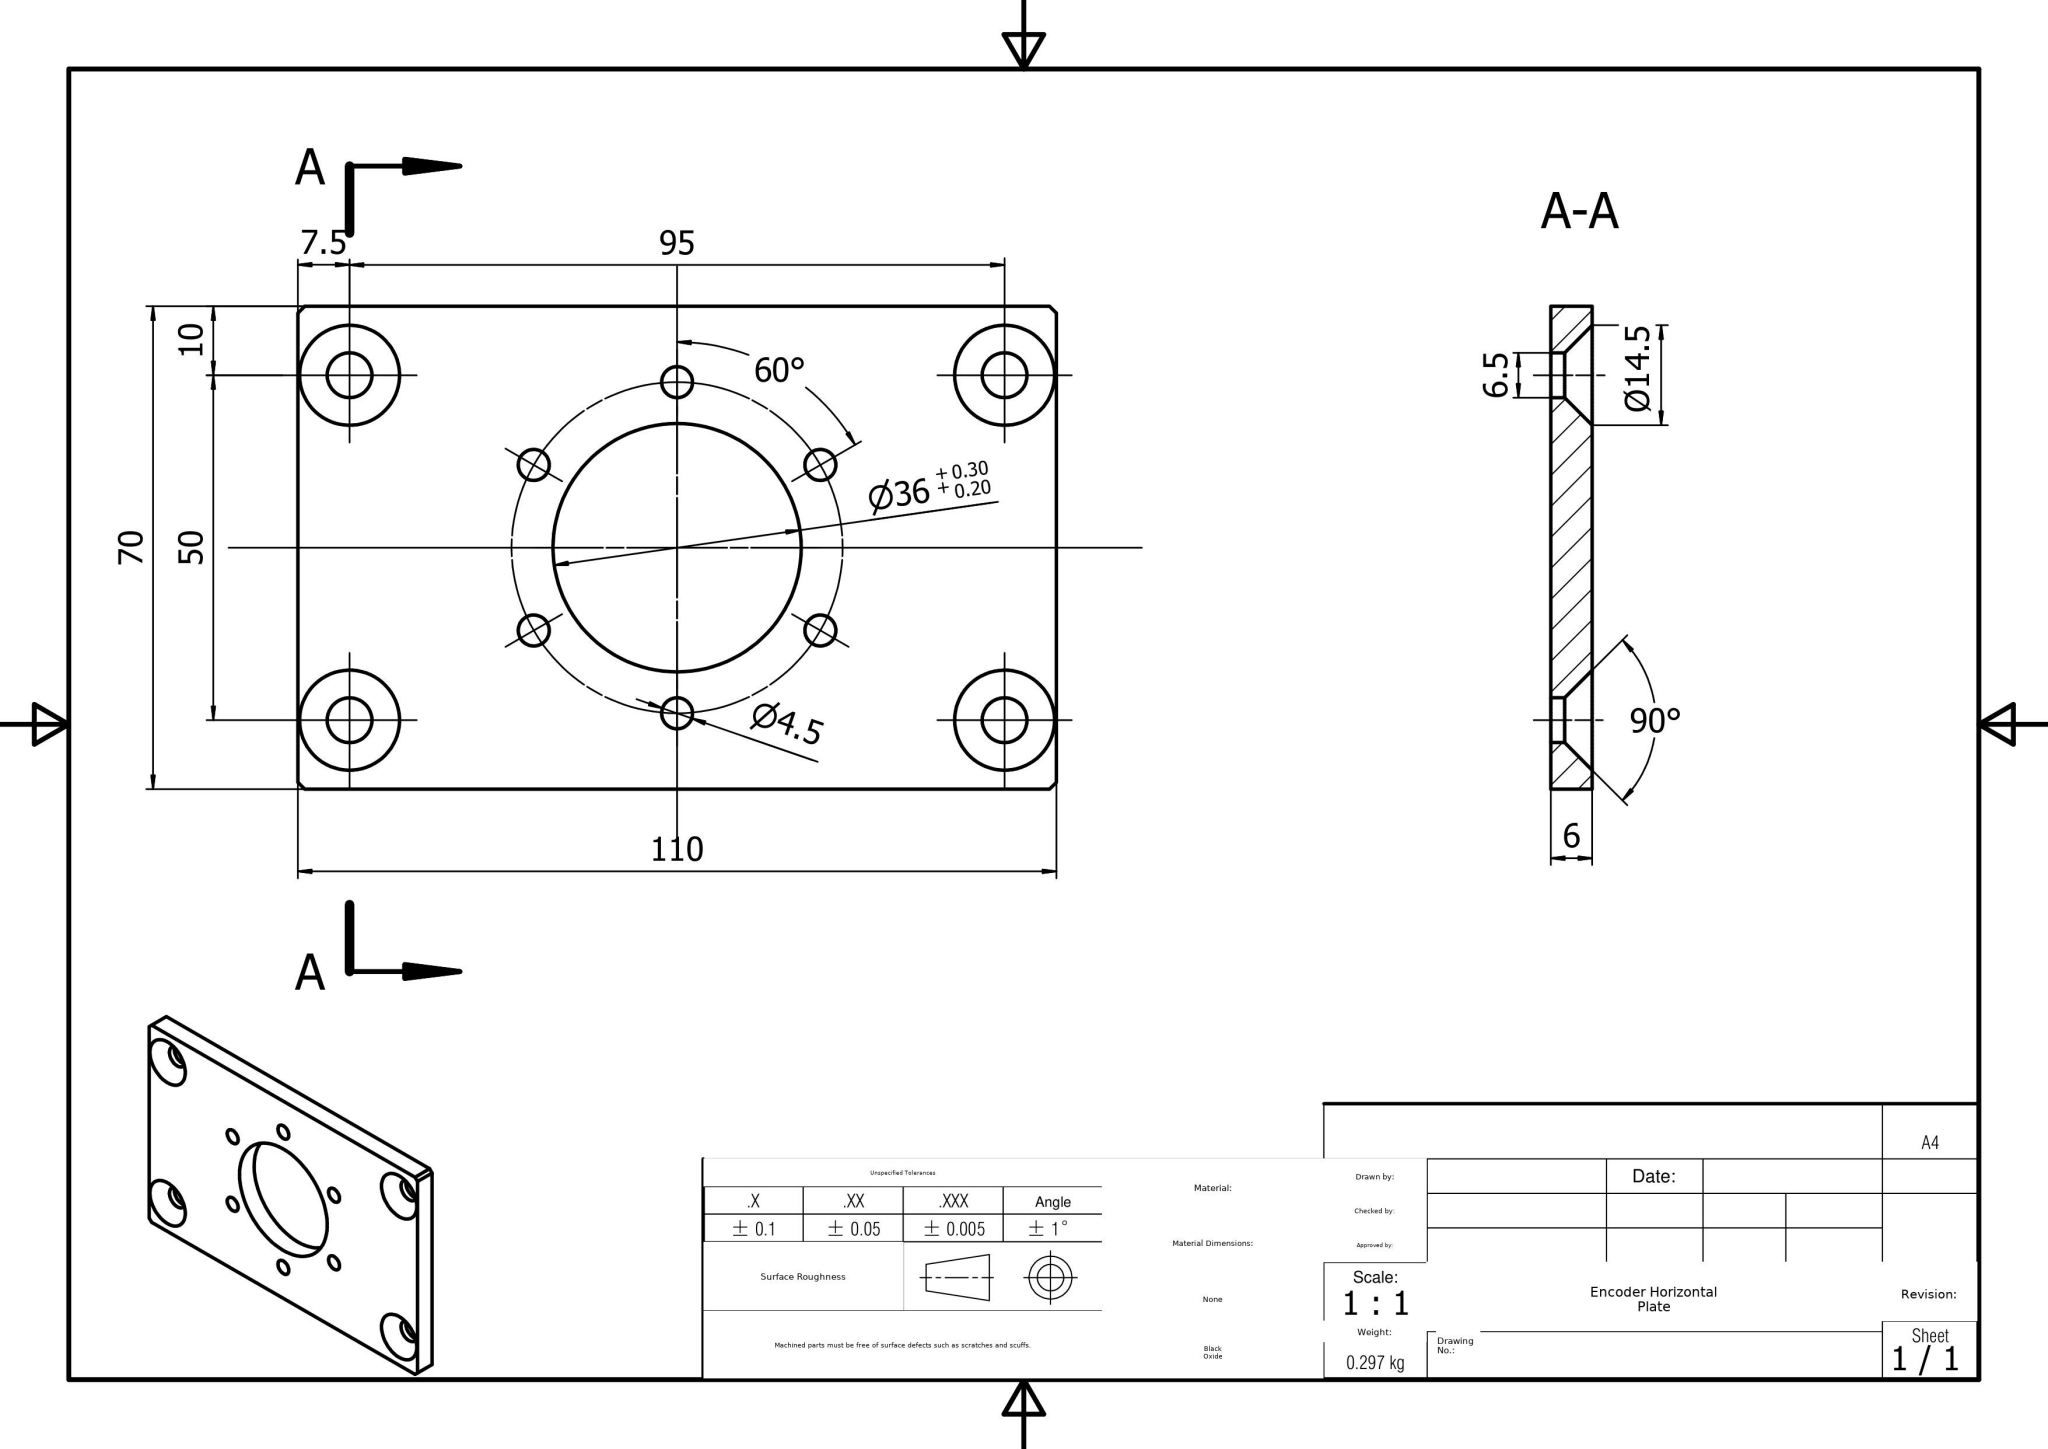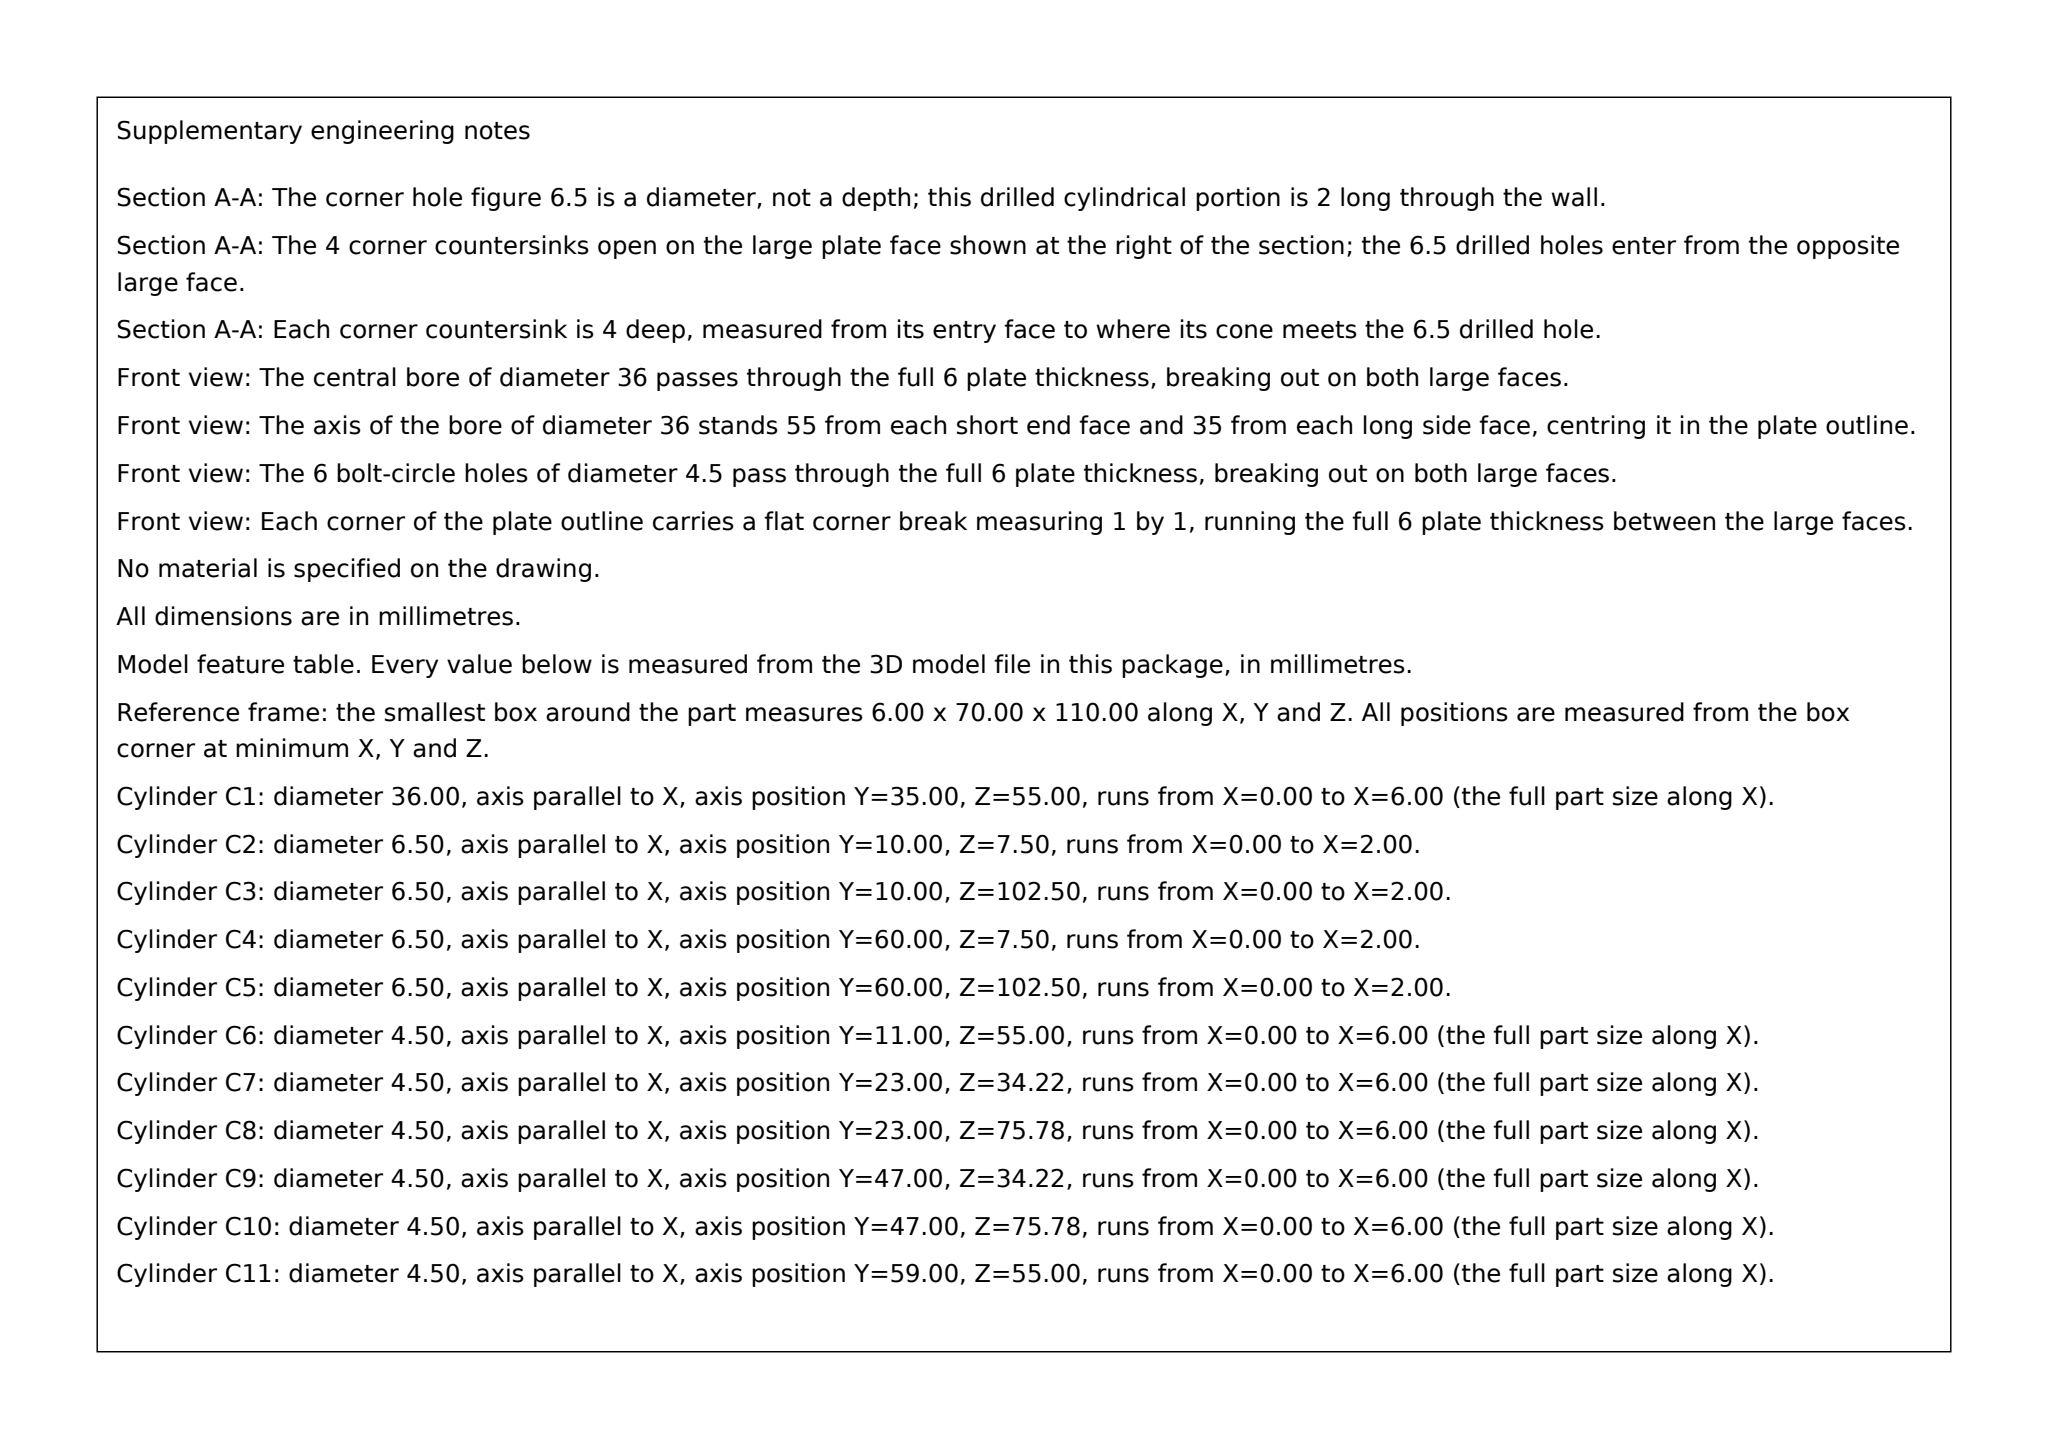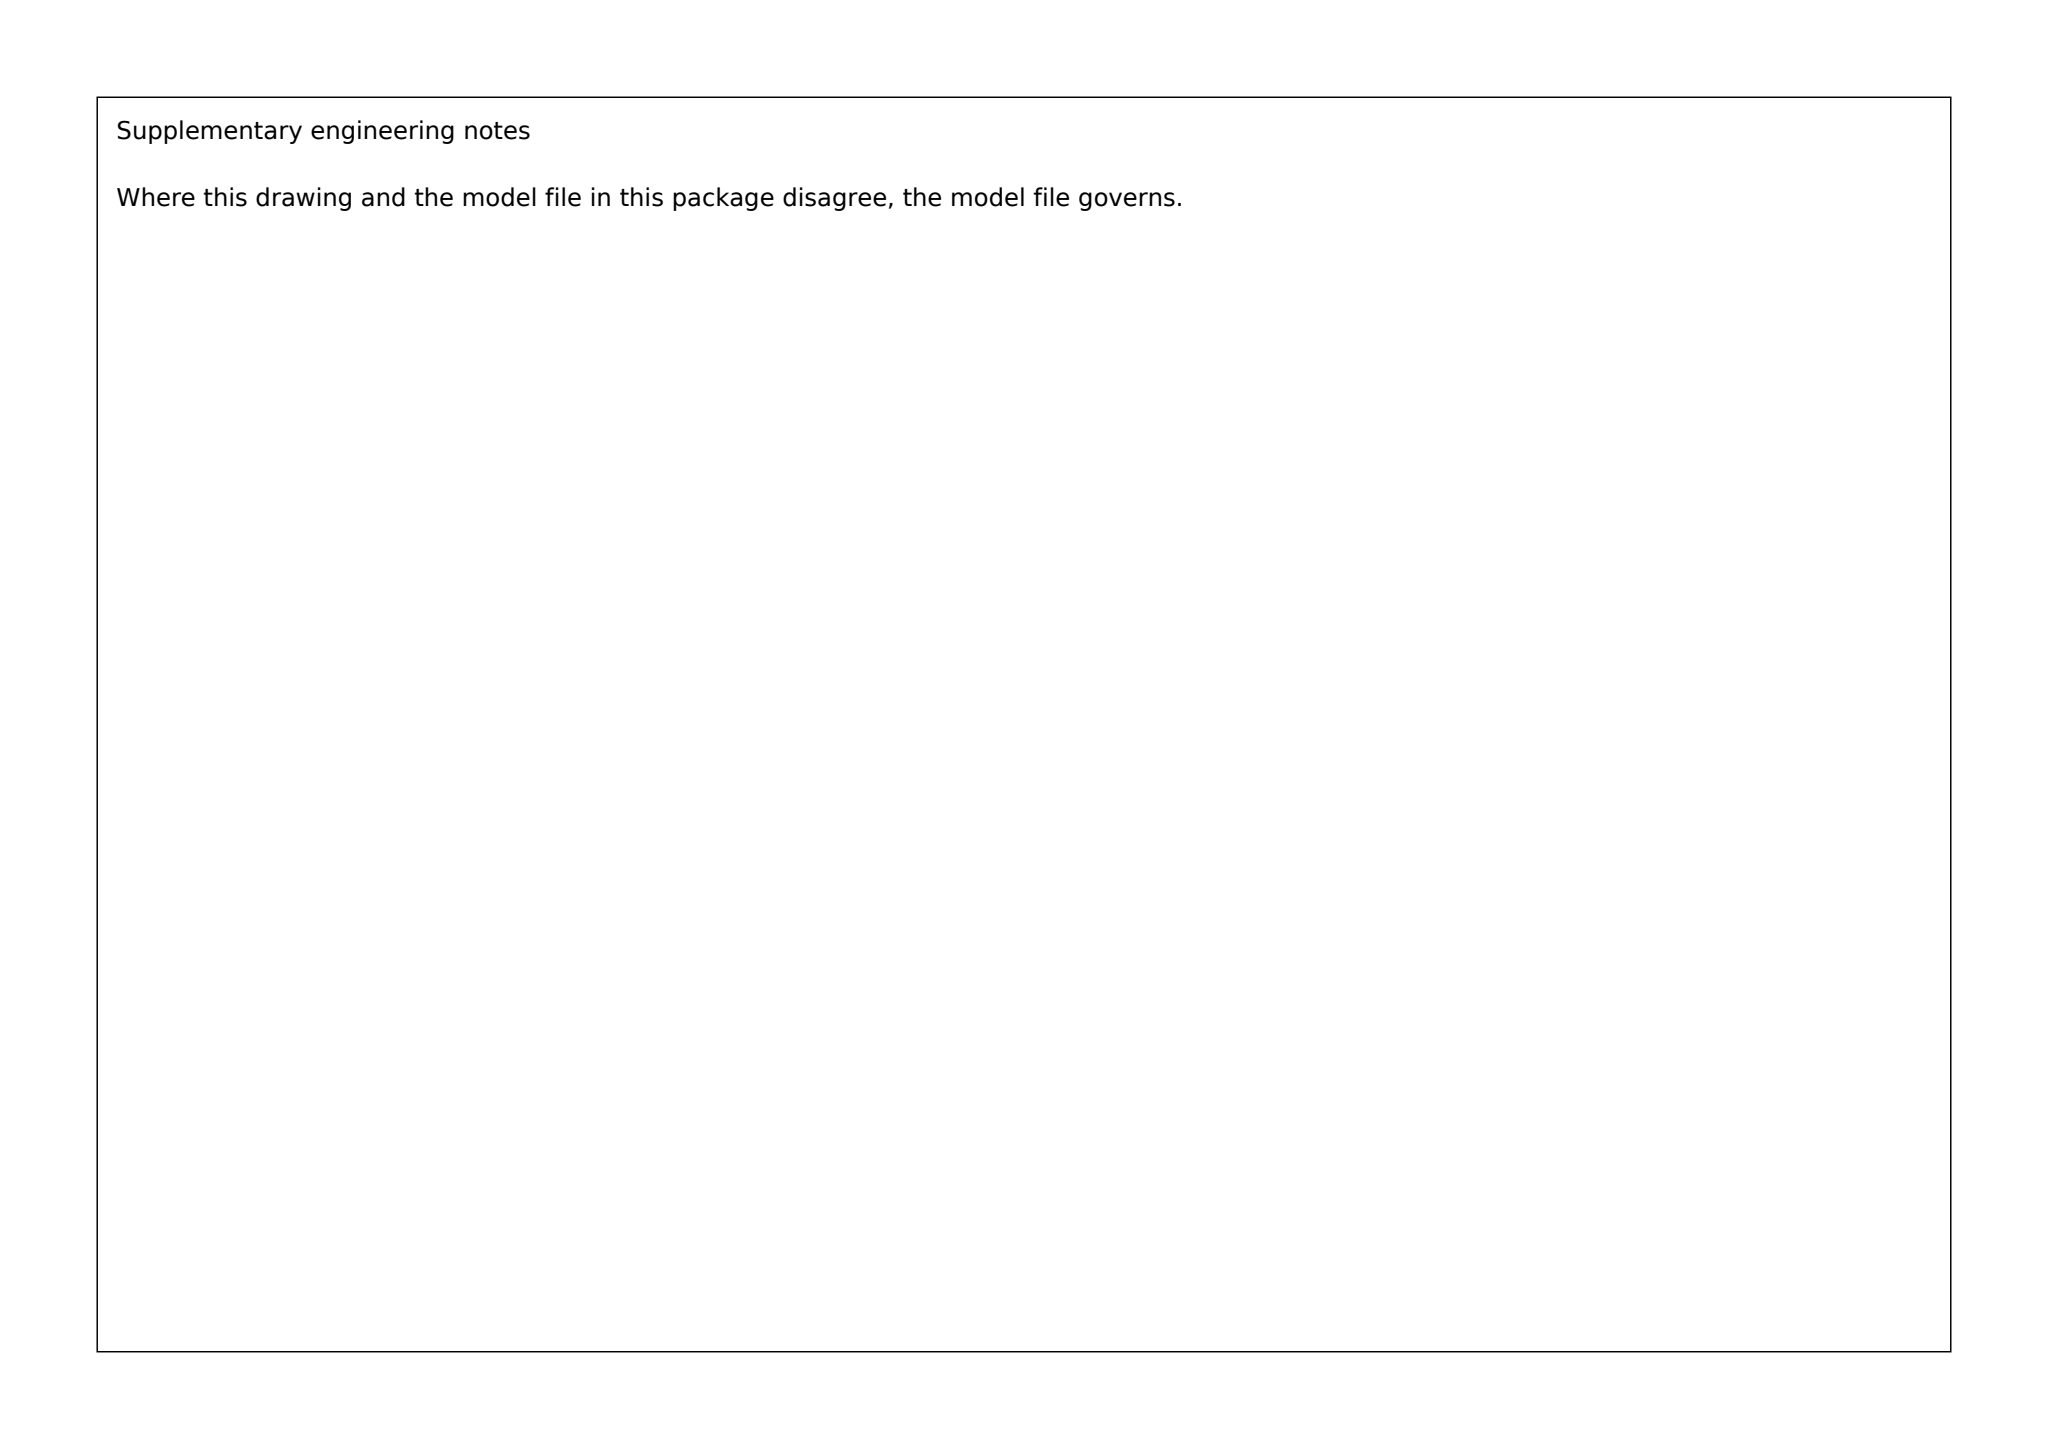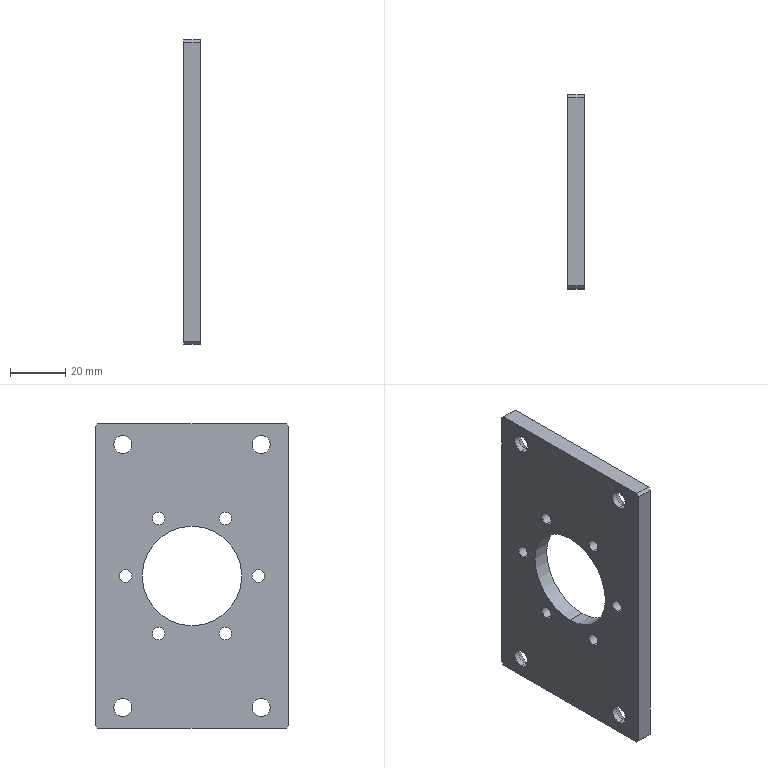Part | SolidWorks | mm | 1 solid | 40 faces | box 6 x 70 x 110 mm | volume 37790 mm3 | cylinder 22 | plane 10 | cone 8 | commonest cylinder face diameters 4.5 x12 6.5 x8 36 x2
Drawing notes:
6X Ø4.5 EQL SP ON Ø48 B.C., CTR'D ON Ø36 BORE | from the solid: Six Ø4.5 holes at (y,z)=(11,55),(23,34.22),(23,75.78),(47,34.22),(47,75.78),(59,55); center (35,55) = Ø36 bore axis; radius 24.00 -> PCD Ø48